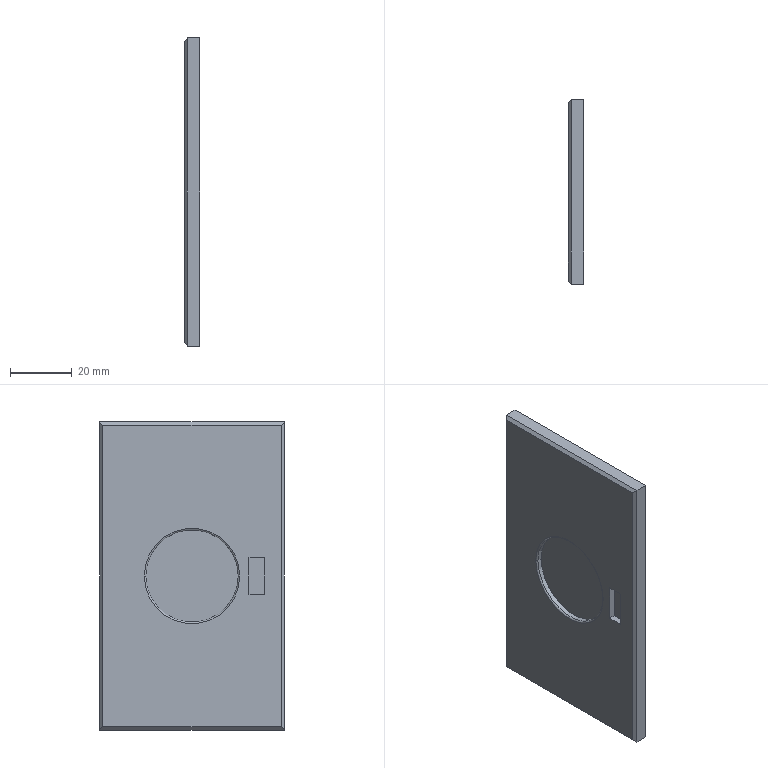Component | SolidWorks | CameraFillLightBracketTable-1 | 1 solid | 20 faces | box 5 x 60 x 100 mm | volume 28303 mm3 | plane 16 | torus 2 | cylinder 2 | commonest cylinder face diameters 30 x2
build123d program:
from build123d import *

# Parameters (mm, degrees)
SKETCH1_W           = 100
SKETCH1_H           = 60
BOSS_EXTRUDE1_DEPTH = 5
CHAMFER1_SIZE       = 1
SKETCH2_R           = 15
CUT_EXTRUDE1_DEPTH  = 2
FILLET1_R           = 0.5
SKETCH3_W           = 12
SKETCH3_H           = 5
CUT_EXTRUDE2_DEPTH  = 2


with BuildPart() as part:
    # Sketch1 → Boss-Extrude1 (new body)
    with BuildSketch(Plane(origin=(0, 0, 0), x_dir=(1, 0, 0), z_dir=(0, 1, 0))):
        Rectangle(SKETCH1_W, SKETCH1_H)
    extrude(amount=BOSS_EXTRUDE1_DEPTH)

    # Chamfer1
    chamfer1_edges = [part.edges().sort_by_distance(p)[0] for p in [
        (-50, 5, 0),
        (0, 5, 30),
        (50, 5, 0),
        (0, 5, -30),
    ]]
    chamfer(chamfer1_edges, length=CHAMFER1_SIZE)

    # Sketch2 → Cut-Extrude1 (cut)
    with BuildSketch(Plane(origin=(0, 5, 0), x_dir=(1, 0, 0), z_dir=(0, 1, 0))):
        with Locations(Location((0, 0, 0), (0, 0, 270))):
            Circle(SKETCH2_R)
    extrude(amount=-CUT_EXTRUDE1_DEPTH, mode=Mode.SUBTRACT)

    # Fillet1
    fillet1_edges = [part.edges().sort_by_distance(p)[0] for p in [
        (0, 5, -15),
    ]]
    fillet(fillet1_edges, radius=FILLET1_R)

    # Sketch3 → Cut-Extrude2 (cut)
    with BuildSketch(Plane(origin=(0, 5, 0), x_dir=(1, 0, 0), z_dir=(0, 1, 0))):
        with Locations((0, -21)):
            Rectangle(SKETCH3_W, SKETCH3_H)
    extrude(amount=-CUT_EXTRUDE2_DEPTH, mode=Mode.SUBTRACT)


solid = part.part

# Placed as in the assembly
solid = solid.moved(Location((298.5, 600, 0), (90, 0, 90)))
STEP:
#1=CARTESIAN_POINT('',(11.555,24.232,-0.));
#2=VERTEX_POINT('',#1);
#3=CARTESIAN_POINT('',(11.555,23.012,-0.));
#4=VERTEX_POINT('',#3);
#5=CARTESIAN_POINT('',(11.555,23.622,-0.));
#6=DIRECTION('',(1.,0.,0.));
#7=DIRECTION('',(0.,-1.,-0.));
#8=AXIS2_PLACEMENT_3D('',#5,#6,#7);
#9=CIRCLE('',#8,0.6102);
#10=EDGE_CURVE('',#2,#4,#9,.T.);
#11=ORIENTED_EDGE('',*,*,#10,.F.);
#12=CARTESIAN_POINT('',(11.575,24.213,-0.));
#13=VERTEX_POINT('',#12);
#14=CARTESIAN_POINT('',(11.575,24.232,-0.));
#15=DIRECTION('',(-0.,-0.,1.));
#16=DIRECTION('',(0.,-1.,-0.));
#17=AXIS2_PLACEMENT_3D('',#14,#15,#16);
#18=CIRCLE('',#17,0.01969);
#19=EDGE_CURVE('',#2,#13,#18,.T.);
#20=ORIENTED_EDGE('',*,*,#19,.T.);
#21=CARTESIAN_POINT('',(11.575,23.031,-0.));
#22=VERTEX_POINT('',#21);
#23=CARTESIAN_POINT('',(11.575,23.622,-0.));
#24=DIRECTION('',(-1.,0.,-0.));
#25=DIRECTION('',(0.,-1.,-0.));
#26=AXIS2_PLACEMENT_3D('',#23,#24,#25);
#27=CIRCLE('',#26,0.5906);
#28=EDGE_CURVE('',#22,#13,#27,.T.);
#29=ORIENTED_EDGE('',*,*,#28,.F.);
#30=CARTESIAN_POINT('',(11.575,23.012,-0.));
#31=DIRECTION('',(0.,0.,-1.));
#32=DIRECTION('',(0.,1.,0.));
#33=AXIS2_PLACEMENT_3D('',#30,#31,#32);
#34=CIRCLE('',#33,0.01969);
#35=EDGE_CURVE('',#4,#22,#34,.T.);
#36=ORIENTED_EDGE('',*,*,#35,.F.);
#37=EDGE_LOOP('',(#11,#20,#29,#36));
#38=FACE_OUTER_BOUND('',#37,.T.);
#39=CARTESIAN_POINT('',(11.575,23.622,-0.));
#40=DIRECTION('',(-1.,0.,-0.));
#41=DIRECTION('',(0.,-1.,-0.));
#42=AXIS2_PLACEMENT_3D('',#39,#40,#41);
#43=TOROIDAL_SURFACE('',#42,0.6102,0.01969);
#44=ADVANCED_FACE('',(#38),#43,.T.);
#45=CARTESIAN_POINT('',(11.634,24.213,-0.));
#46=VERTEX_POINT('',#45);
#47=CARTESIAN_POINT('',(11.634,23.031,-0.));
#48=VERTEX_POINT('',#47);
#49=CARTESIAN_POINT('',(11.634,23.622,-0.));
#50=DIRECTION('',(-1.,0.,-0.));
#51=DIRECTION('',(0.,-1.,-0.));
#52=AXIS2_PLACEMENT_3D('',#49,#50,#51);
#53=CIRCLE('',#52,0.5906);
#54=EDGE_CURVE('',#46,#48,#53,.T.);
#55=ORIENTED_EDGE('',*,*,#54,.F.);
#56=CARTESIAN_POINT('',(11.634,24.213,-0.));
#57=DIRECTION('',(-1.,0.,-0.));
#58=VECTOR('',#57,39.37);
#59=LINE('',#56,#58);
#60=EDGE_CURVE('',#46,#13,#59,.T.);
#61=ORIENTED_EDGE('',*,*,#60,.T.);
#62=CARTESIAN_POINT('',(11.575,23.622,-0.));
#63=DIRECTION('',(-1.,0.,-0.));
#64=DIRECTION('',(0.,-1.,-0.));
#65=AXIS2_PLACEMENT_3D('',#62,#63,#64);
#66=CIRCLE('',#65,0.5906);
#67=EDGE_CURVE('',#13,#22,#66,.T.);
#68=ORIENTED_EDGE('',*,*,#67,.T.);
#69=CARTESIAN_POINT('',(11.634,23.031,-0.));
#70=DIRECTION('',(-1.,0.,-0.));
#71=VECTOR('',#70,39.37);
#72=LINE('',#69,#71);
#73=EDGE_CURVE('',#48,#22,#72,.T.);
#74=ORIENTED_EDGE('',*,*,#73,.F.);
#75=EDGE_LOOP('',(#55,#61,#68,#74));
#76=FACE_OUTER_BOUND('',#75,.T.);
#77=CARTESIAN_POINT('',(11.634,23.622,-0.));
#78=DIRECTION('',(-1.,0.,-0.));
#79=DIRECTION('',(0.,-1.,-0.));
#80=AXIS2_PLACEMENT_3D('',#77,#78,#79);
#81=CYLINDRICAL_SURFACE('',#80,0.5906);
#82=ADVANCED_FACE('',(#76),#81,.F.);
#83=CARTESIAN_POINT('',(11.594,24.803,1.969));
#84=VERTEX_POINT('',#83);
#85=CARTESIAN_POINT('',(11.752,24.803,1.969));
#86=VERTEX_POINT('',#85);
#87=CARTESIAN_POINT('',(11.555,24.803,1.969));
#88=DIRECTION('',(1.,0.,0.));
#89=VECTOR('',#88,39.37);
#90=LINE('',#87,#89);
#91=EDGE_CURVE('',#84,#86,#90,.T.);
#92=ORIENTED_EDGE('',*,*,#91,.F.);
#93=CARTESIAN_POINT('',(11.594,22.441,1.969));
#94=VERTEX_POINT('',#93);
#95=CARTESIAN_POINT('',(11.594,22.441,1.969));
#96=DIRECTION('',(0.,-1.,0.));
#97=VECTOR('',#96,39.37);
#98=LINE('',#95,#97);
#99=EDGE_CURVE('',#84,#94,#98,.T.);
#100=ORIENTED_EDGE('',*,*,#99,.T.);
#101=CARTESIAN_POINT('',(11.752,22.441,1.969));
#102=VERTEX_POINT('',#101);
#103=CARTESIAN_POINT('',(11.555,22.441,1.969));
#104=DIRECTION('',(1.,0.,0.));
#105=VECTOR('',#104,39.37);
#106=LINE('',#103,#105);
#107=EDGE_CURVE('',#94,#102,#106,.T.);
#108=ORIENTED_EDGE('',*,*,#107,.T.);
#109=CARTESIAN_POINT('',(11.752,24.803,1.969));
#110=DIRECTION('',(-0.,1.,-0.));
#111=VECTOR('',#110,39.37);
#112=LINE('',#109,#111);
#113=EDGE_CURVE('',#102,#86,#112,.T.);
#114=ORIENTED_EDGE('',*,*,#113,.T.);
#115=EDGE_LOOP('',(#92,#100,#108,#114));
#116=FACE_OUTER_BOUND('',#115,.T.);
#117=CARTESIAN_POINT('',(11.555,24.803,1.969));
#118=DIRECTION('',(0.,-0.,-1.));
#119=DIRECTION('',(0.,-1.,0.));
#120=AXIS2_PLACEMENT_3D('',#117,#118,#119);
#121=PLANE('',#120);
#122=ADVANCED_FACE('',(#116),#121,.F.);
#123=CARTESIAN_POINT('',(11.594,24.803,-1.969));
#124=VERTEX_POINT('',#123);
#125=CARTESIAN_POINT('',(11.752,24.803,-1.969));
#126=VERTEX_POINT('',#125);
#127=CARTESIAN_POINT('',(11.555,24.803,-1.969));
#128=DIRECTION('',(1.,0.,0.));
#129=VECTOR('',#128,39.37);
#130=LINE('',#127,#129);
#131=EDGE_CURVE('',#124,#126,#130,.T.);
#132=ORIENTED_EDGE('',*,*,#131,.F.);
#133=CARTESIAN_POINT('',(11.594,24.803,1.969));
#134=DIRECTION('',(-0.,-0.,1.));
#135=VECTOR('',#134,39.37);
#136=LINE('',#133,#135);
#137=EDGE_CURVE('',#124,#84,#136,.T.);
#138=ORIENTED_EDGE('',*,*,#137,.T.);
#139=ORIENTED_EDGE('',*,*,#91,.T.);
#140=CARTESIAN_POINT('',(11.752,24.803,-1.969));
#141=DIRECTION('',(0.,0.,-1.));
#142=VECTOR('',#141,39.37);
#143=LINE('',#140,#142);
#144=EDGE_CURVE('',#86,#126,#143,.T.);
#145=ORIENTED_EDGE('',*,*,#144,.T.);
#146=EDGE_LOOP('',(#132,#138,#139,#145));
#147=FACE_OUTER_BOUND('',#146,.T.);
#148=CARTESIAN_POINT('',(11.555,24.803,-1.969));
#149=DIRECTION('',(0.,-1.,-0.));
#150=DIRECTION('',(-0.,-0.,1.));
#151=AXIS2_PLACEMENT_3D('',#148,#149,#150);
#152=PLANE('',#151);
#153=ADVANCED_FACE('',(#147),#152,.F.);
#154=CARTESIAN_POINT('',(11.594,22.441,-1.969));
#155=VERTEX_POINT('',#154);
#156=CARTESIAN_POINT('',(11.752,22.441,-1.969));
#157=VERTEX_POINT('',#156);
#158=CARTESIAN_POINT('',(11.555,22.441,-1.969));
#159=DIRECTION('',(1.,0.,0.));
#160=VECTOR('',#159,39.37);
#161=LINE('',#158,#160);
#162=EDGE_CURVE('',#155,#157,#161,.T.);
#163=ORIENTED_EDGE('',*,*,#162,.F.);
#164=CARTESIAN_POINT('',(11.594,24.803,-1.969));
#165=DIRECTION('',(-0.,1.,-0.));
#166=VECTOR('',#165,39.37);
#167=LINE('',#164,#166);
#168=EDGE_CURVE('',#155,#124,#167,.T.);
#169=ORIENTED_EDGE('',*,*,#168,.T.);
#170=ORIENTED_EDGE('',*,*,#131,.T.);
#171=CARTESIAN_POINT('',(11.752,24.803,-1.969));
#172=DIRECTION('',(0.,-1.,0.));
#173=VECTOR('',#172,39.37);
#174=LINE('',#171,#173);
#175=EDGE_CURVE('',#126,#157,#174,.T.);
#176=ORIENTED_EDGE('',*,*,#175,.T.);
#177=EDGE_LOOP('',(#163,#169,#170,#176));
#178=FACE_OUTER_BOUND('',#177,.T.);
#179=CARTESIAN_POINT('',(11.555,24.803,-1.969));
#180=DIRECTION('',(-0.,0.,1.));
#181=DIRECTION('',(-0.,1.,-0.));
#182=AXIS2_PLACEMENT_3D('',#179,#180,#181);
#183=PLANE('',#182);
#184=ADVANCED_FACE('',(#178),#183,.F.);
#185=ORIENTED_EDGE('',*,*,#107,.F.);
#186=CARTESIAN_POINT('',(11.594,22.441,-1.969));
#187=DIRECTION('',(0.,0.,-1.));
#188=VECTOR('',#187,39.37);
#189=LINE('',#186,#188);
#190=EDGE_CURVE('',#94,#155,#189,.T.);
#191=ORIENTED_EDGE('',*,*,#190,.T.);
#192=ORIENTED_EDGE('',*,*,#162,.T.);
#193=CARTESIAN_POINT('',(11.752,22.441,-1.969));
#194=DIRECTION('',(-0.,-0.,1.));
#195=VECTOR('',#194,39.37);
#196=LINE('',#193,#195);
#197=EDGE_CURVE('',#157,#102,#196,.T.);
#198=ORIENTED_EDGE('',*,*,#197,.T.);
#199=EDGE_LOOP('',(#185,#191,#192,#198));
#200=FACE_OUTER_BOUND('',#199,.T.);
#201=CARTESIAN_POINT('',(11.555,22.441,-1.969));
#202=DIRECTION('',(-0.,1.,0.));
#203=DIRECTION('',(0.,0.,-1.));
#204=AXIS2_PLACEMENT_3D('',#201,#202,#203);
#205=PLANE('',#204);
#206=ADVANCED_FACE('',(#200),#205,.F.);
#207=CARTESIAN_POINT('',(11.555,22.697,0.2362));
#208=VERTEX_POINT('',#207);
#209=CARTESIAN_POINT('',(11.555,22.894,0.2362));
#210=VERTEX_POINT('',#209);
#211=CARTESIAN_POINT('',(11.555,22.894,0.2362));
#212=DIRECTION('',(-0.,1.,-0.));
#213=VECTOR('',#212,39.37);
#214=LINE('',#211,#213);
#215=EDGE_CURVE('',#208,#210,#214,.T.);
#216=ORIENTED_EDGE('',*,*,#215,.F.);
#217=CARTESIAN_POINT('',(11.555,22.697,-0.2362));
#218=VERTEX_POINT('',#217);
#219=CARTESIAN_POINT('',(11.555,22.697,-0.2362));
#220=DIRECTION('',(-0.,-0.,1.));
#221=VECTOR('',#220,39.37);
#222=LINE('',#219,#221);
#223=EDGE_CURVE('',#218,#208,#222,.T.);
#224=ORIENTED_EDGE('',*,*,#223,.F.);
#225=CARTESIAN_POINT('',(11.555,22.894,-0.2362));
#226=VERTEX_POINT('',#225);
#227=CARTESIAN_POINT('',(11.555,22.894,-0.2362));
#228=DIRECTION('',(0.,-1.,0.));
#229=VECTOR('',#228,39.37);
#230=LINE('',#227,#229);
#231=EDGE_CURVE('',#226,#218,#230,.T.);
#232=ORIENTED_EDGE('',*,*,#231,.F.);
#233=CARTESIAN_POINT('',(11.555,22.894,-0.2362));
#234=DIRECTION('',(0.,0.,-1.));
#235=VECTOR('',#234,39.37);
#236=LINE('',#233,#235);
#237=EDGE_CURVE('',#210,#226,#236,.T.);
#238=ORIENTED_EDGE('',*,*,#237,.F.);
#239=EDGE_LOOP('',(#216,#224,#232,#238));
#240=FACE_BOUND('',#239,.T.);
#241=CARTESIAN_POINT('',(11.555,23.622,-0.));
#242=DIRECTION('',(1.,0.,0.));
#243=DIRECTION('',(0.,-1.,-0.));
#244=AXIS2_PLACEMENT_3D('',#241,#242,#243);
#245=CIRCLE('',#244,0.6102);
#246=EDGE_CURVE('',#4,#2,#245,.T.);
#247=ORIENTED_EDGE('',*,*,#246,.T.);
#248=ORIENTED_EDGE('',*,*,#10,.T.);
#249=EDGE_LOOP('',(#247,#248));
#250=FACE_BOUND('',#249,.T.);
#251=CARTESIAN_POINT('',(11.555,24.764,-1.929));
#252=VERTEX_POINT('',#251);
#253=CARTESIAN_POINT('',(11.555,22.48,-1.929));
#254=VERTEX_POINT('',#253);
#255=CARTESIAN_POINT('',(11.555,22.441,-1.929));
#256=DIRECTION('',(0.,-1.,0.));
#257=VECTOR('',#256,39.37);
#258=LINE('',#255,#257);
#259=EDGE_CURVE('',#252,#254,#258,.T.);
#260=ORIENTED_EDGE('',*,*,#259,.T.);
#261=CARTESIAN_POINT('',(11.555,22.48,1.929));
#262=VERTEX_POINT('',#261);
#263=CARTESIAN_POINT('',(11.555,22.48,1.969));
#264=DIRECTION('',(-0.,-0.,1.));
#265=VECTOR('',#264,39.37);
#266=LINE('',#263,#265);
#267=EDGE_CURVE('',#254,#262,#266,.T.);
#268=ORIENTED_EDGE('',*,*,#267,.T.);
#269=CARTESIAN_POINT('',(11.555,24.764,1.929));
#270=VERTEX_POINT('',#269);
#271=CARTESIAN_POINT('',(11.555,24.803,1.929));
#272=DIRECTION('',(-0.,1.,-0.));
#273=VECTOR('',#272,39.37);
#274=LINE('',#271,#273);
#275=EDGE_CURVE('',#262,#270,#274,.T.);
#276=ORIENTED_EDGE('',*,*,#275,.T.);
#277=CARTESIAN_POINT('',(11.555,24.764,-1.969));
#278=DIRECTION('',(0.,0.,-1.));
#279=VECTOR('',#278,39.37);
#280=LINE('',#277,#279);
#281=EDGE_CURVE('',#270,#252,#280,.T.);
#282=ORIENTED_EDGE('',*,*,#281,.T.);
#283=EDGE_LOOP('',(#260,#268,#276,#282));
#284=FACE_OUTER_BOUND('',#283,.T.);
#285=CARTESIAN_POINT('',(11.555,23.622,-0.));
#286=DIRECTION('',(-1.,-0.,-0.));
#287=DIRECTION('',(0.,-1.,-0.));
#288=AXIS2_PLACEMENT_3D('',#285,#286,#287);
#289=PLANE('',#288);
#290=ADVANCED_FACE('',(#240,#250,#284),#289,.T.);
#291=ORIENTED_EDGE('',*,*,#113,.F.);
#292=ORIENTED_EDGE('',*,*,#197,.F.);
#293=ORIENTED_EDGE('',*,*,#175,.F.);
#294=ORIENTED_EDGE('',*,*,#144,.F.);
#295=EDGE_LOOP('',(#291,#292,#293,#294));
#296=FACE_OUTER_BOUND('',#295,.T.);
#297=CARTESIAN_POINT('',(11.752,23.622,-0.));
#298=DIRECTION('',(-1.,-0.,-0.));
#299=DIRECTION('',(0.,-1.,-0.));
#300=AXIS2_PLACEMENT_3D('',#297,#298,#299);
#301=PLANE('',#300);
#302=ADVANCED_FACE('',(#296),#301,.F.);
#303=CARTESIAN_POINT('',(11.175,24.383,1.549));
#304=DIRECTION('',(-0.5774,-0.5774,-0.5774));
#305=VECTOR('',#304,39.37);
#306=LINE('',#303,#305);
#307=EDGE_CURVE('',#84,#270,#306,.T.);
#308=ORIENTED_EDGE('',*,*,#307,.F.);
#309=ORIENTED_EDGE('',*,*,#137,.F.);
#310=CARTESIAN_POINT('',(10.912,24.121,-1.286));
#311=DIRECTION('',(0.5774,0.5774,-0.5774));
#312=VECTOR('',#311,39.37);
#313=LINE('',#310,#312);
#314=EDGE_CURVE('',#252,#124,#313,.T.);
#315=ORIENTED_EDGE('',*,*,#314,.F.);
#316=ORIENTED_EDGE('',*,*,#281,.F.);
#317=EDGE_LOOP('',(#308,#309,#315,#316));
#318=FACE_OUTER_BOUND('',#317,.T.);
#319=CARTESIAN_POINT('',(11.555,24.764,-0.));
#320=DIRECTION('',(-0.7071,0.7071,0.));
#321=DIRECTION('',(-0.,-0.,1.));
#322=AXIS2_PLACEMENT_3D('',#319,#320,#321);
#323=PLANE('',#322);
#324=ADVANCED_FACE('',(#318),#323,.T.);
#325=ORIENTED_EDGE('',*,*,#314,.T.);
#326=ORIENTED_EDGE('',*,*,#168,.F.);
#327=CARTESIAN_POINT('',(11.175,22.861,-1.549));
#328=DIRECTION('',(0.5774,-0.5774,-0.5774));
#329=VECTOR('',#328,39.37);
#330=LINE('',#327,#329);
#331=EDGE_CURVE('',#254,#155,#330,.T.);
#332=ORIENTED_EDGE('',*,*,#331,.F.);
#333=ORIENTED_EDGE('',*,*,#259,.F.);
#334=EDGE_LOOP('',(#325,#326,#332,#333));
#335=FACE_OUTER_BOUND('',#334,.T.);
#336=CARTESIAN_POINT('',(11.555,23.622,-1.929));
#337=DIRECTION('',(-0.7071,-0.,-0.7071));
#338=DIRECTION('',(-0.,1.,-0.));
#339=AXIS2_PLACEMENT_3D('',#336,#337,#338);
#340=PLANE('',#339);
#341=ADVANCED_FACE('',(#335),#340,.T.);
#342=ORIENTED_EDGE('',*,*,#307,.T.);
#343=ORIENTED_EDGE('',*,*,#275,.F.);
#344=CARTESIAN_POINT('',(11.175,22.861,1.549));
#345=DIRECTION('',(-0.5774,0.5774,-0.5774));
#346=VECTOR('',#345,39.37);
#347=LINE('',#344,#346);
#348=EDGE_CURVE('',#94,#262,#347,.T.);
#349=ORIENTED_EDGE('',*,*,#348,.F.);
#350=ORIENTED_EDGE('',*,*,#99,.F.);
#351=EDGE_LOOP('',(#342,#343,#349,#350));
#352=FACE_OUTER_BOUND('',#351,.T.);
#353=CARTESIAN_POINT('',(11.555,23.622,1.929));
#354=DIRECTION('',(-0.7071,0.,0.7071));
#355=DIRECTION('',(0.,-1.,0.));
#356=AXIS2_PLACEMENT_3D('',#353,#354,#355);
#357=PLANE('',#356);
#358=ADVANCED_FACE('',(#352),#357,.T.);
#359=ORIENTED_EDGE('',*,*,#331,.T.);
#360=ORIENTED_EDGE('',*,*,#190,.F.);
#361=ORIENTED_EDGE('',*,*,#348,.T.);
#362=ORIENTED_EDGE('',*,*,#267,.F.);
#363=EDGE_LOOP('',(#359,#360,#361,#362));
#364=FACE_OUTER_BOUND('',#363,.T.);
#365=CARTESIAN_POINT('',(11.555,22.48,-0.));
#366=DIRECTION('',(-0.7071,-0.7071,-0.));
#367=DIRECTION('',(0.,0.,-1.));
#368=AXIS2_PLACEMENT_3D('',#365,#366,#367);
#369=PLANE('',#368);
#370=ADVANCED_FACE('',(#364),#369,.T.);
#371=ORIENTED_EDGE('',*,*,#60,.F.);
#372=CARTESIAN_POINT('',(11.634,23.622,-0.));
#373=DIRECTION('',(-1.,0.,-0.));
#374=DIRECTION('',(0.,-1.,-0.));
#375=AXIS2_PLACEMENT_3D('',#372,#373,#374);
#376=CIRCLE('',#375,0.5906);
#377=EDGE_CURVE('',#48,#46,#376,.T.);
#378=ORIENTED_EDGE('',*,*,#377,.F.);
#379=ORIENTED_EDGE('',*,*,#73,.T.);
#380=ORIENTED_EDGE('',*,*,#28,.T.);
#381=EDGE_LOOP('',(#371,#378,#379,#380));
#382=FACE_OUTER_BOUND('',#381,.T.);
#383=CARTESIAN_POINT('',(11.634,23.622,-0.));
#384=DIRECTION('',(-1.,0.,-0.));
#385=DIRECTION('',(0.,-1.,-0.));
#386=AXIS2_PLACEMENT_3D('',#383,#384,#385);
#387=CYLINDRICAL_SURFACE('',#386,0.5906);
#388=ADVANCED_FACE('',(#382),#387,.F.);
#389=ORIENTED_EDGE('',*,*,#377,.T.);
#390=ORIENTED_EDGE('',*,*,#54,.T.);
#391=EDGE_LOOP('',(#389,#390));
#392=FACE_OUTER_BOUND('',#391,.T.);
#393=CARTESIAN_POINT('',(11.634,23.622,-0.));
#394=DIRECTION('',(-1.,-0.,-0.));
#395=DIRECTION('',(0.,-1.,-0.));
#396=AXIS2_PLACEMENT_3D('',#393,#394,#395);
#397=PLANE('',#396);
#398=ADVANCED_FACE('',(#392),#397,.T.);
#399=ORIENTED_EDGE('',*,*,#19,.F.);
#400=ORIENTED_EDGE('',*,*,#246,.F.);
#401=ORIENTED_EDGE('',*,*,#35,.T.);
#402=ORIENTED_EDGE('',*,*,#67,.F.);
#403=EDGE_LOOP('',(#399,#400,#401,#402));
#404=FACE_OUTER_BOUND('',#403,.T.);
#405=CARTESIAN_POINT('',(11.575,23.622,-0.));
#406=DIRECTION('',(-1.,0.,-0.));
#407=DIRECTION('',(0.,-1.,-0.));
#408=AXIS2_PLACEMENT_3D('',#405,#406,#407);
#409=TOROIDAL_SURFACE('',#408,0.6102,0.01969);
#410=ADVANCED_FACE('',(#404),#409,.T.);
#411=ORIENTED_EDGE('',*,*,#215,.T.);
#412=CARTESIAN_POINT('',(11.634,22.894,0.2362));
#413=VERTEX_POINT('',#412);
#414=CARTESIAN_POINT('',(11.634,22.894,0.2362));
#415=DIRECTION('',(-1.,0.,-0.));
#416=VECTOR('',#415,39.37);
#417=LINE('',#414,#416);
#418=EDGE_CURVE('',#413,#210,#417,.T.);
#419=ORIENTED_EDGE('',*,*,#418,.F.);
#420=CARTESIAN_POINT('',(11.634,22.697,0.2362));
#421=VERTEX_POINT('',#420);
#422=CARTESIAN_POINT('',(11.634,22.894,0.2362));
#423=DIRECTION('',(-0.,1.,-0.));
#424=VECTOR('',#423,39.37);
#425=LINE('',#422,#424);
#426=EDGE_CURVE('',#421,#413,#425,.T.);
#427=ORIENTED_EDGE('',*,*,#426,.F.);
#428=CARTESIAN_POINT('',(11.634,22.697,0.2362));
#429=DIRECTION('',(-1.,0.,-0.));
#430=VECTOR('',#429,39.37);
#431=LINE('',#428,#430);
#432=EDGE_CURVE('',#421,#208,#431,.T.);
#433=ORIENTED_EDGE('',*,*,#432,.T.);
#434=EDGE_LOOP('',(#411,#419,#427,#433));
#435=FACE_OUTER_BOUND('',#434,.T.);
#436=CARTESIAN_POINT('',(11.634,22.894,0.2362));
#437=DIRECTION('',(-0.,0.,1.));
#438=DIRECTION('',(-0.,1.,-0.));
#439=AXIS2_PLACEMENT_3D('',#436,#437,#438);
#440=PLANE('',#439);
#441=ADVANCED_FACE('',(#435),#440,.F.);
#442=ORIENTED_EDGE('',*,*,#223,.T.);
#443=ORIENTED_EDGE('',*,*,#432,.F.);
#444=CARTESIAN_POINT('',(11.634,22.697,-0.2362));
#445=VERTEX_POINT('',#444);
#446=CARTESIAN_POINT('',(11.634,22.697,-0.2362));
#447=DIRECTION('',(-0.,-0.,1.));
#448=VECTOR('',#447,39.37);
#449=LINE('',#446,#448);
#450=EDGE_CURVE('',#445,#421,#449,.T.);
#451=ORIENTED_EDGE('',*,*,#450,.F.);
#452=CARTESIAN_POINT('',(11.634,22.697,-0.2362));
#453=DIRECTION('',(-1.,0.,-0.));
#454=VECTOR('',#453,39.37);
#455=LINE('',#452,#454);
#456=EDGE_CURVE('',#445,#218,#455,.T.);
#457=ORIENTED_EDGE('',*,*,#456,.T.);
#458=EDGE_LOOP('',(#442,#443,#451,#457));
#459=FACE_OUTER_BOUND('',#458,.T.);
#460=CARTESIAN_POINT('',(11.634,22.697,-0.2362));
#461=DIRECTION('',(0.,-1.,-0.));
#462=DIRECTION('',(-0.,-0.,1.));
#463=AXIS2_PLACEMENT_3D('',#460,#461,#462);
#464=PLANE('',#463);
#465=ADVANCED_FACE('',(#459),#464,.F.);
#466=ORIENTED_EDGE('',*,*,#231,.T.);
#467=ORIENTED_EDGE('',*,*,#456,.F.);
#468=CARTESIAN_POINT('',(11.634,22.894,-0.2362));
#469=VERTEX_POINT('',#468);
#470=CARTESIAN_POINT('',(11.634,22.894,-0.2362));
#471=DIRECTION('',(0.,-1.,0.));
#472=VECTOR('',#471,39.37);
#473=LINE('',#470,#472);
#474=EDGE_CURVE('',#469,#445,#473,.T.);
#475=ORIENTED_EDGE('',*,*,#474,.F.);
#476=CARTESIAN_POINT('',(11.634,22.894,-0.2362));
#477=DIRECTION('',(-1.,0.,-0.));
#478=VECTOR('',#477,39.37);
#479=LINE('',#476,#478);
#480=EDGE_CURVE('',#469,#226,#479,.T.);
#481=ORIENTED_EDGE('',*,*,#480,.T.);
#482=EDGE_LOOP('',(#466,#467,#475,#481));
#483=FACE_OUTER_BOUND('',#482,.T.);
#484=CARTESIAN_POINT('',(11.634,22.894,-0.2362));
#485=DIRECTION('',(0.,-0.,-1.));
#486=DIRECTION('',(0.,-1.,0.));
#487=AXIS2_PLACEMENT_3D('',#484,#485,#486);
#488=PLANE('',#487);
#489=ADVANCED_FACE('',(#483),#488,.F.);
#490=ORIENTED_EDGE('',*,*,#237,.T.);
#491=ORIENTED_EDGE('',*,*,#480,.F.);
#492=CARTESIAN_POINT('',(11.634,22.894,-0.2362));
#493=DIRECTION('',(0.,0.,-1.));
#494=VECTOR('',#493,39.37);
#495=LINE('',#492,#494);
#496=EDGE_CURVE('',#413,#469,#495,.T.);
#497=ORIENTED_EDGE('',*,*,#496,.F.);
#498=ORIENTED_EDGE('',*,*,#418,.T.);
#499=EDGE_LOOP('',(#490,#491,#497,#498));
#500=FACE_OUTER_BOUND('',#499,.T.);
#501=CARTESIAN_POINT('',(11.634,22.894,-0.2362));
#502=DIRECTION('',(-0.,1.,0.));
#503=DIRECTION('',(0.,0.,-1.));
#504=AXIS2_PLACEMENT_3D('',#501,#502,#503);
#505=PLANE('',#504);
#506=ADVANCED_FACE('',(#500),#505,.F.);
#507=ORIENTED_EDGE('',*,*,#426,.T.);
#508=ORIENTED_EDGE('',*,*,#496,.T.);
#509=ORIENTED_EDGE('',*,*,#474,.T.);
#510=ORIENTED_EDGE('',*,*,#450,.T.);
#511=EDGE_LOOP('',(#507,#508,#509,#510));
#512=FACE_OUTER_BOUND('',#511,.T.);
#513=CARTESIAN_POINT('',(11.634,23.622,-0.));
#514=DIRECTION('',(-1.,-0.,-0.));
#515=DIRECTION('',(0.,-1.,-0.));
#516=AXIS2_PLACEMENT_3D('',#513,#514,#515);
#517=PLANE('',#516);
#518=ADVANCED_FACE('',(#512),#517,.T.);
#519=CLOSED_SHELL('',(#44,#82,#122,#153,#184,#206,#290,#302,#324,#341,#358,#370,#388,#398,#410,#441,#465,#489,#506,#518));
#520=MANIFOLD_SOLID_BREP('',#519);
#521=CARTESIAN_POINT('',(0.,0.,0.));
#522=DIRECTION('',(0.,0.,1.));
#523=DIRECTION('',(1.,0.,0.));
#524=AXIS2_PLACEMENT_3D('',#521,#522,#523);
#525=(LENGTH_UNIT()NAMED_UNIT(*)SI_UNIT($,.METRE.));
#526=LENGTH_MEASURE_WITH_UNIT(LENGTH_MEASURE(0.0254),#525);
#527=DIMENSIONAL_EXPONENTS(1.,0.,0.,0.,0.,0.,0.);
#528=(CONVERSION_BASED_UNIT('',#526)LENGTH_UNIT()NAMED_UNIT(#527));
#529=UNCERTAINTY_MEASURE_WITH_UNIT(LENGTH_MEASURE(0.00001),#528,'','');
#530=(NAMED_UNIT(*)PLANE_ANGLE_UNIT()SI_UNIT($,.RADIAN.));
#531=(NAMED_UNIT(*)SI_UNIT($,.STERADIAN.)SOLID_ANGLE_UNIT());
#532=(GEOMETRIC_REPRESENTATION_CONTEXT(3)GLOBAL_UNCERTAINTY_ASSIGNED_CONTEXT((#529))GLOBAL_UNIT_ASSIGNED_CONTEXT((#528,#530,#531))REPRESENTATION_CONTEXT('',''));
#533=ADVANCED_BREP_SHAPE_REPRESENTATION('',(#520,#524),#532);
#534=COLOUR_RGB('',0.7922,0.8196,0.9333);
#535=FILL_AREA_STYLE_COLOUR('',#534);
#536=FILL_AREA_STYLE('',(#535));
#537=SURFACE_STYLE_FILL_AREA(#536);
#538=SURFACE_SIDE_STYLE('',(#537));
#539=SURFACE_STYLE_USAGE(.BOTH.,#538);
#540=PRESENTATION_STYLE_ASSIGNMENT((#539));
#541=STYLED_ITEM('',(#540),#520);
#542=(LENGTH_UNIT()NAMED_UNIT(*)SI_UNIT($,.METRE.));
#543=LENGTH_MEASURE_WITH_UNIT(LENGTH_MEASURE(0.0254),#542);
#544=DIMENSIONAL_EXPONENTS(1.,0.,0.,0.,0.,0.,0.);
#545=(CONVERSION_BASED_UNIT('',#543)LENGTH_UNIT()NAMED_UNIT(#544));
#546=UNCERTAINTY_MEASURE_WITH_UNIT(LENGTH_MEASURE(0.00001),#545,'','');
#547=(NAMED_UNIT(*)PLANE_ANGLE_UNIT()SI_UNIT($,.RADIAN.));
#548=(NAMED_UNIT(*)SI_UNIT($,.STERADIAN.)SOLID_ANGLE_UNIT());
#549=(GEOMETRIC_REPRESENTATION_CONTEXT(3)GLOBAL_UNCERTAINTY_ASSIGNED_CONTEXT((#546))GLOBAL_UNIT_ASSIGNED_CONTEXT((#545,#547,#548))REPRESENTATION_CONTEXT('',''));
#550=MECHANICAL_DESIGN_GEOMETRIC_PRESENTATION_REPRESENTATION('',(#541),#549);
#551=PRESENTATION_LAYER_ASSIGNMENT('','',(#541));